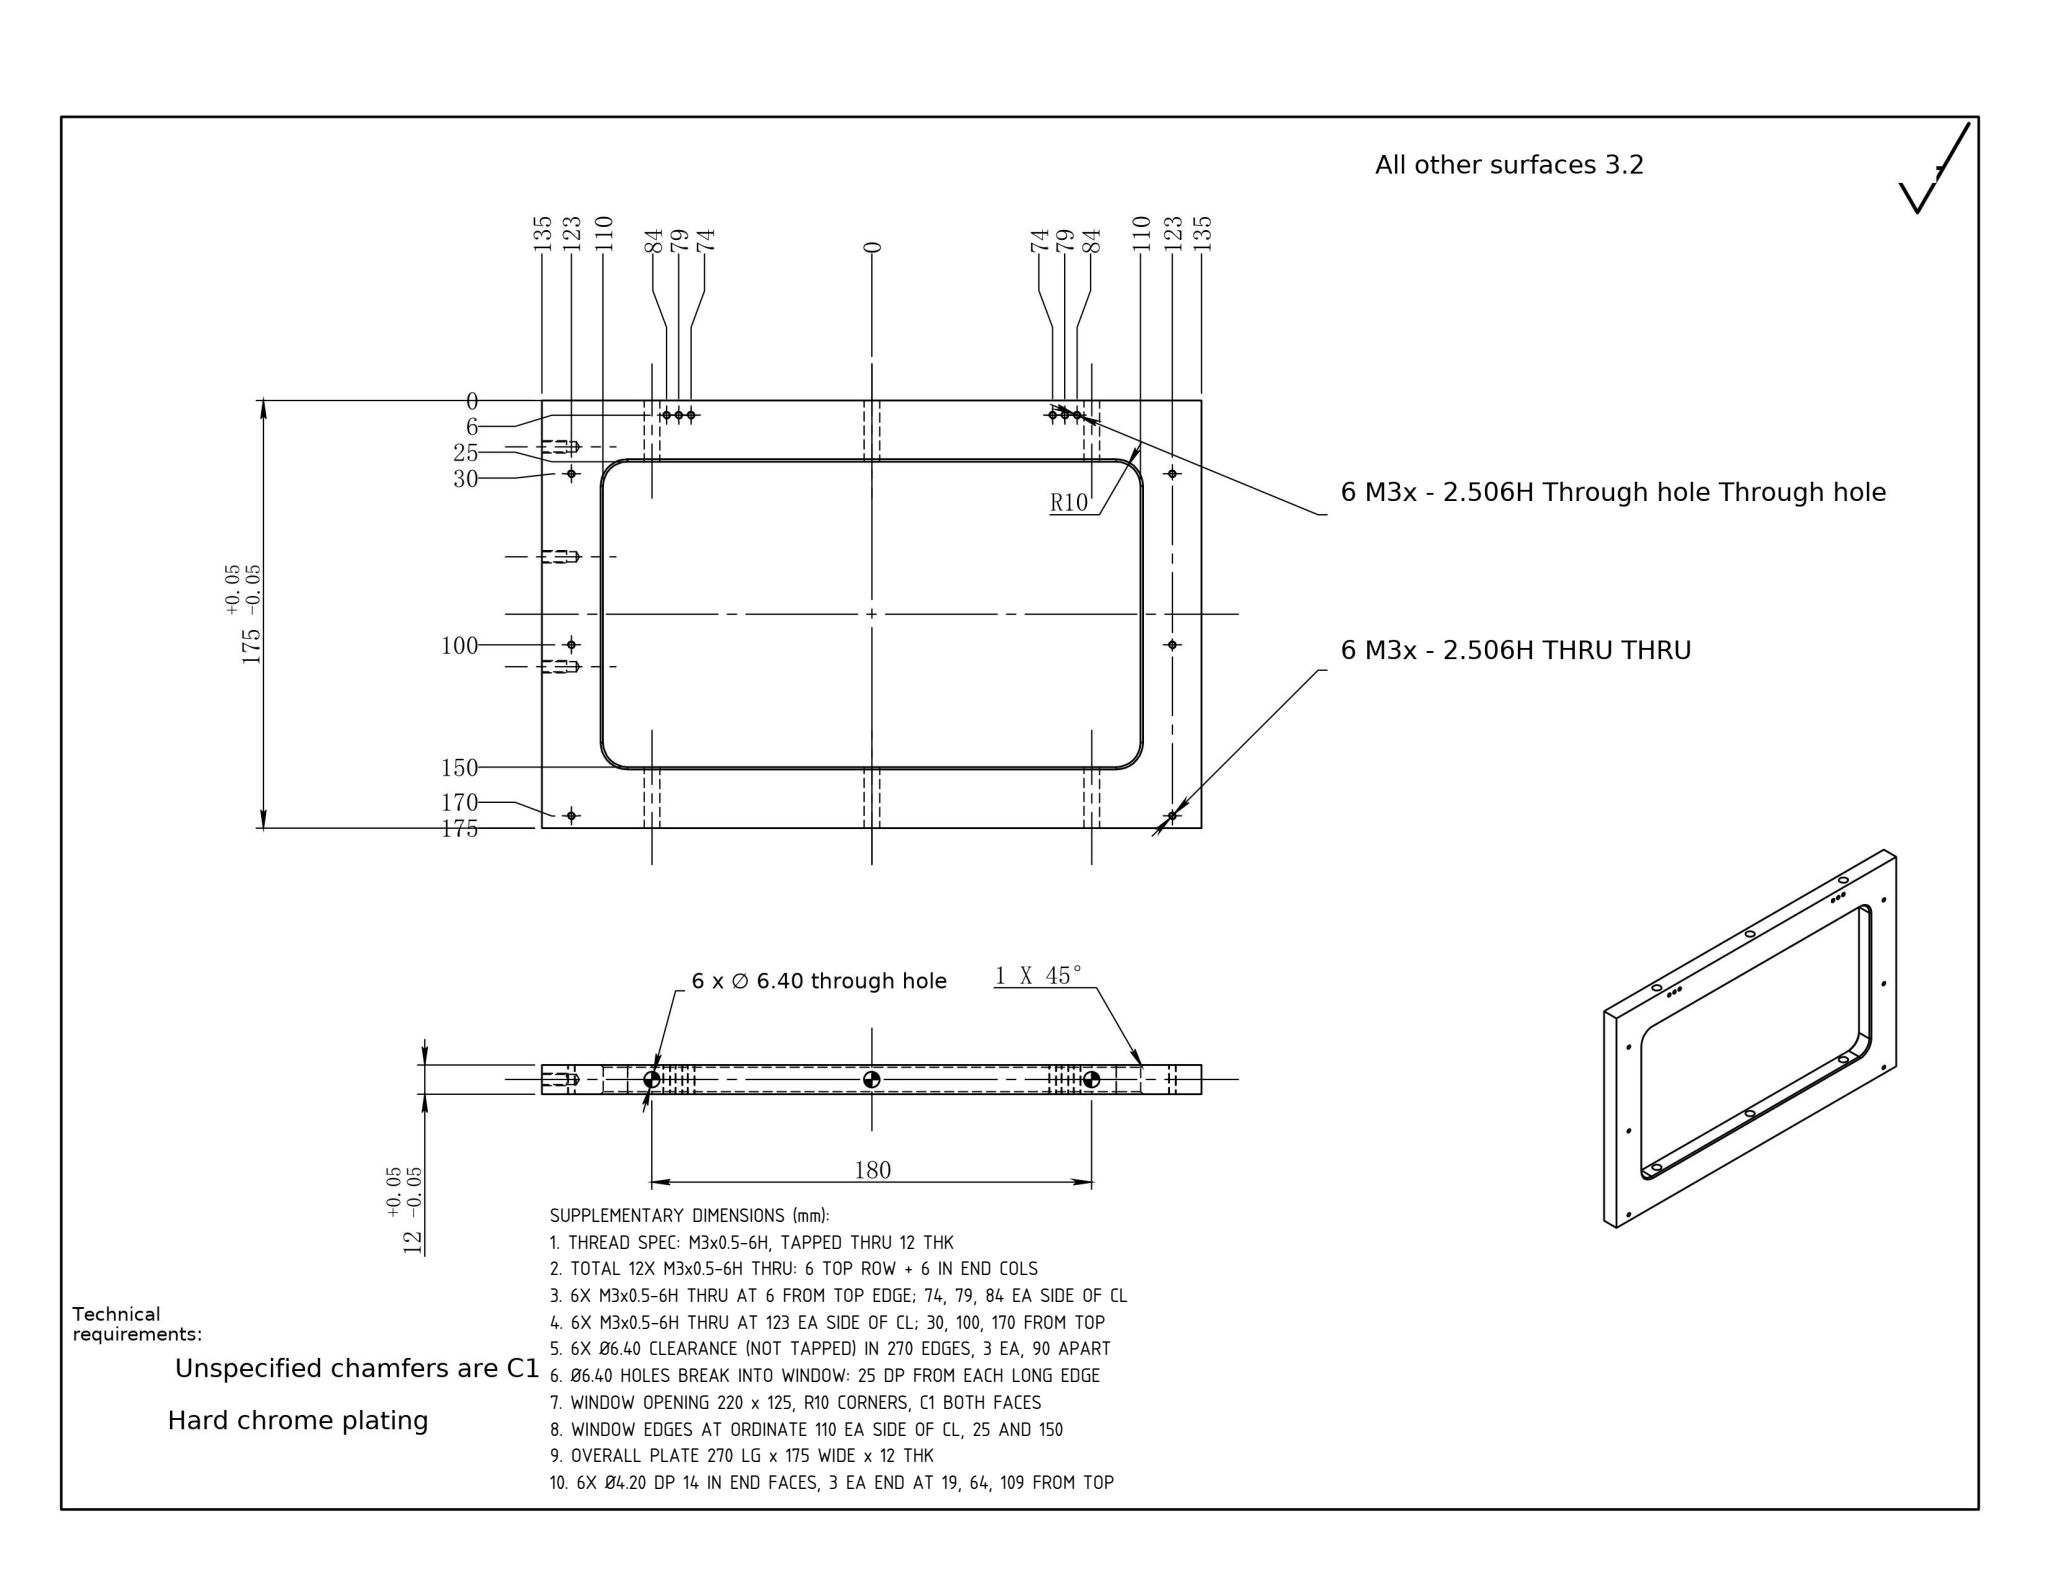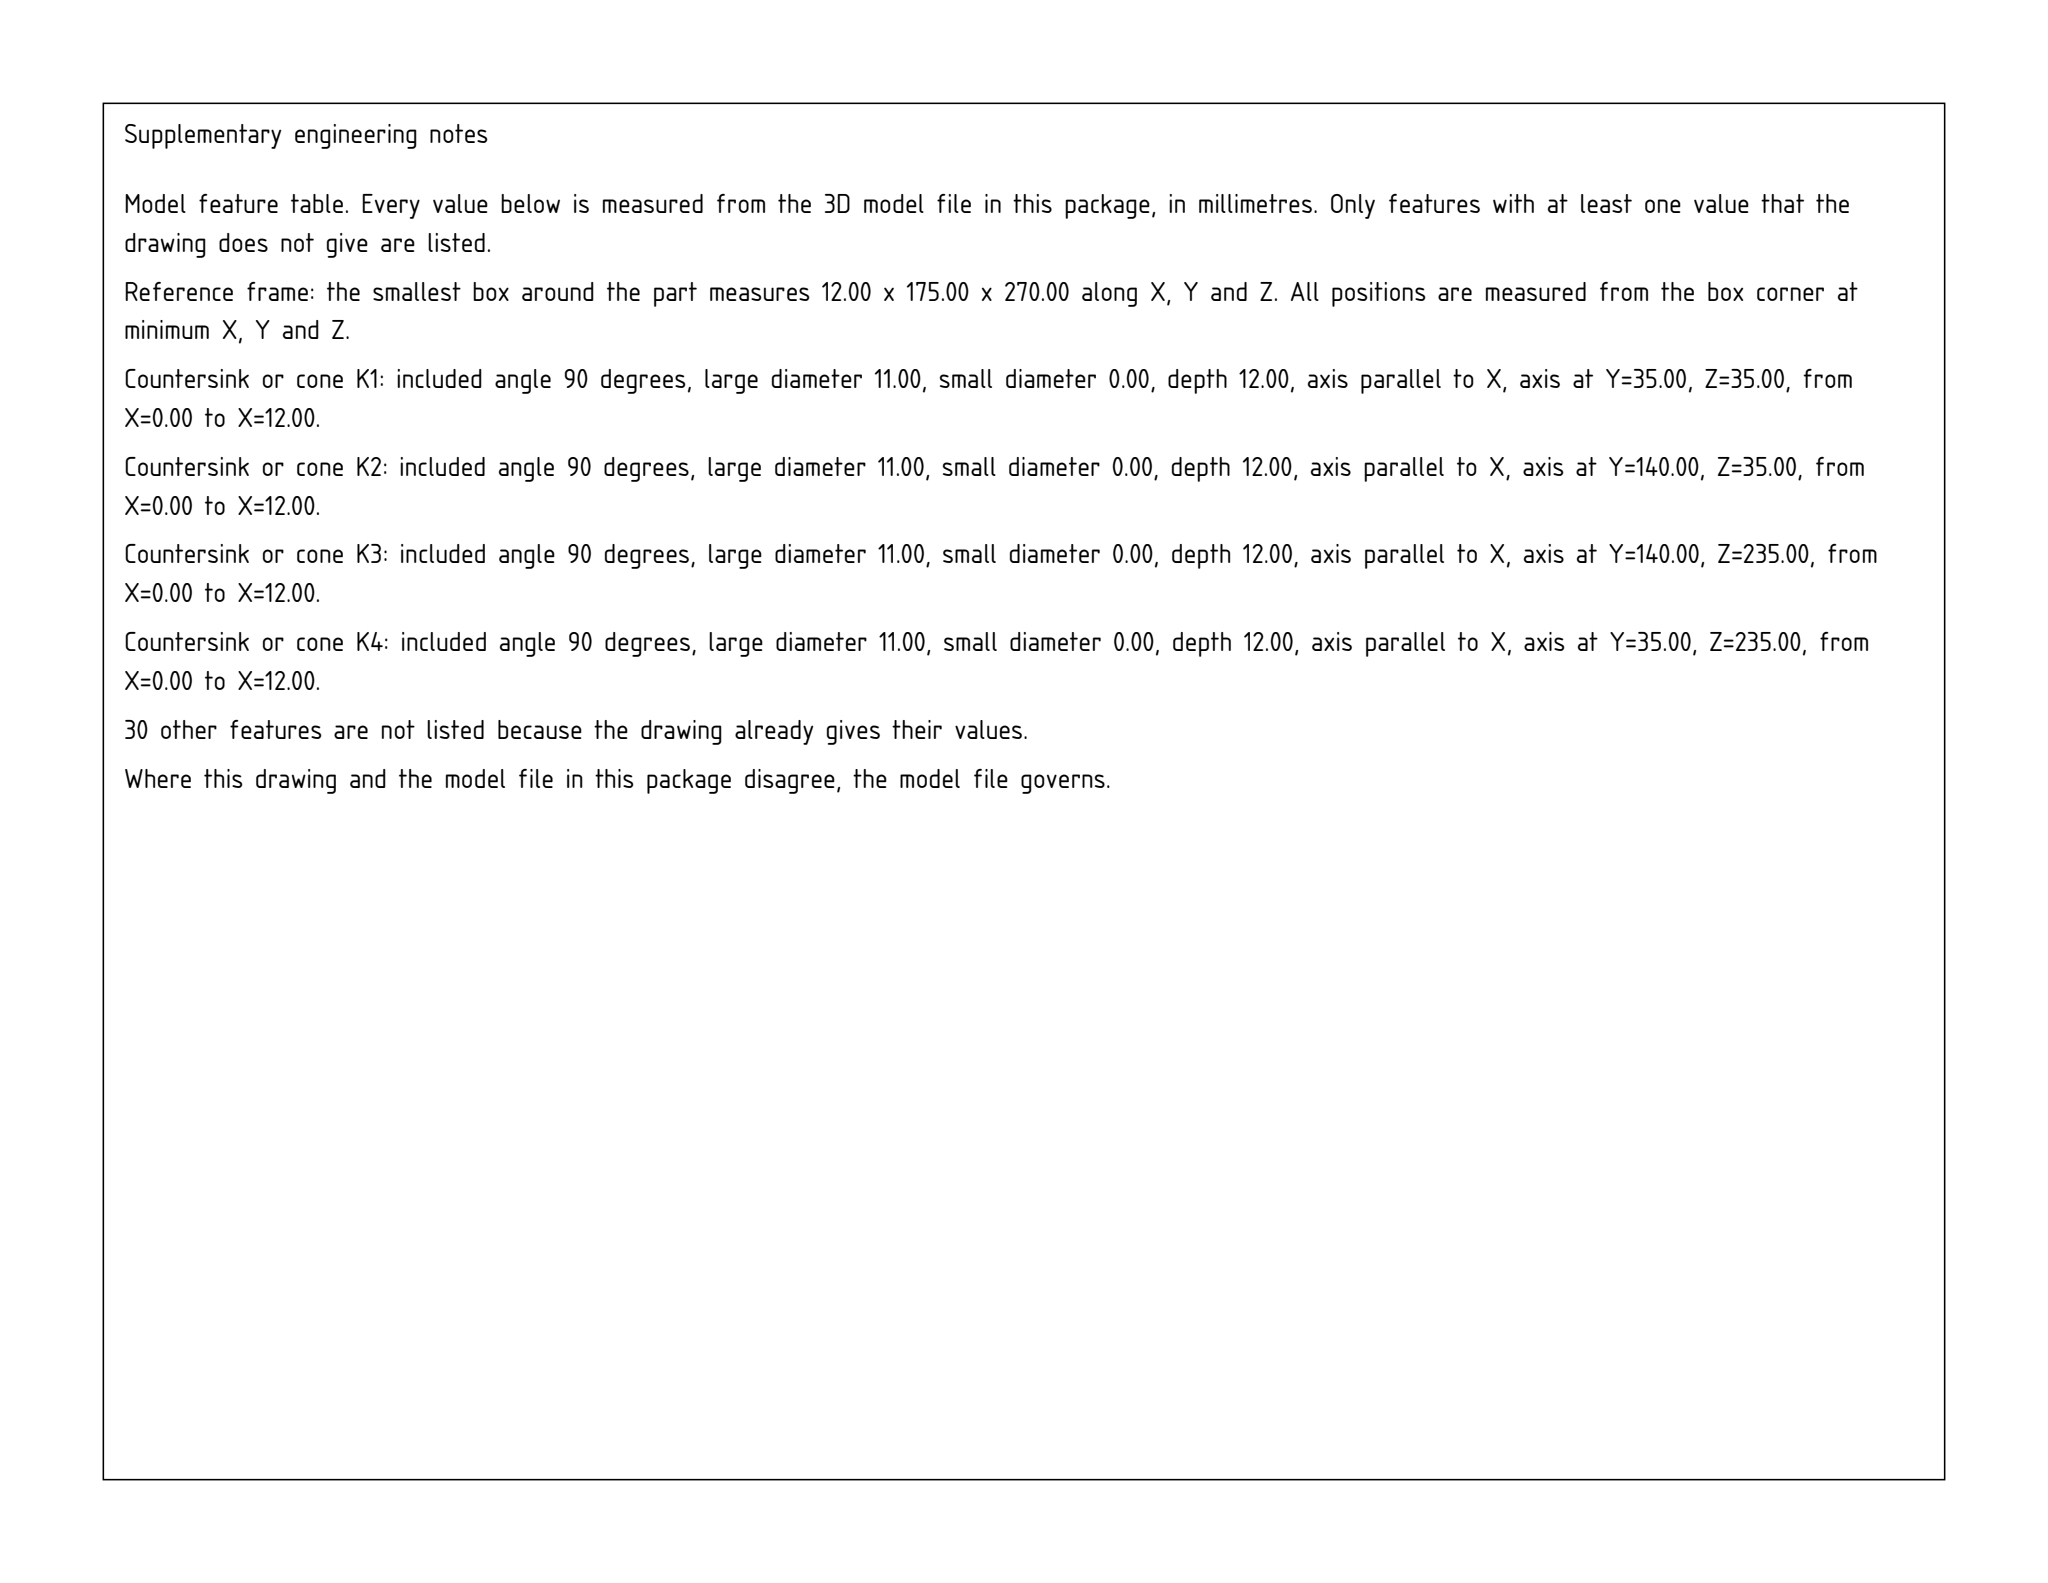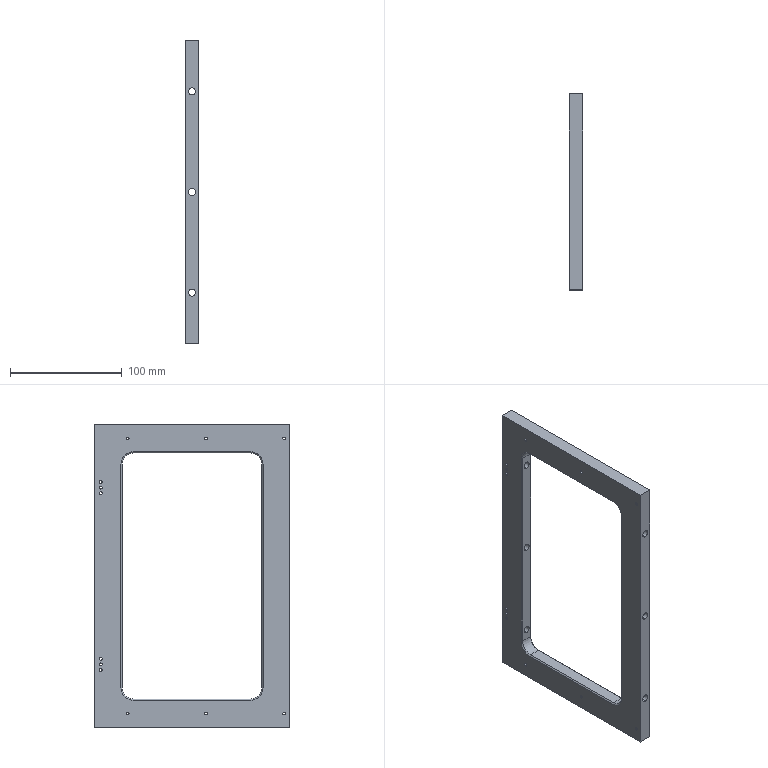Part | SolidWorks | mm | 1 solid | 78 faces | box 12 x 175 x 270 mm | volume 231223 mm3 | cylinder 46 | plane 18 | cone 14 | commonest cylinder face diameters 2.5 x24 6.4 x12 4.2 x6 20 x4
build123d program:
from build123d import *

# Parameters (mm, degrees)
SKETCH1_W                      = 12
SKETCH1_H                      = 270
BOSS_EXTRUDE1_DEPTH            = 87.5
SKETCH2_W                      = 220
SKETCH2_H                      = 125
CUT_EXTRUDE1_DEPTH             = 162.323
F_6_4_6_4_DIAMETER_HOLE1_D     = 6.4
F_6_4_6_4_DIAMETER_HOLE1_DEPTH = 25
FILLET1_R                      = 10
CHAMFER1_SIZE                  = 1
M5_TAPPED_HOLE1_D              = 4.2
M5_TAPPED_HOLE1_DEPTH          = 14
M5_TAPPED_HOLE1_TIP            = 1.262
M3_TAPPED_HOLE2_D              = 2.5
M3_TAPPED_HOLE1_D              = 2.5
LPATTERN1_COUNT                = 3
LPATTERN1_PITCH                = 70
MIRROR2_COPY_1_D               = 2.5
MIRROR2_COPY_2_D               = 2.5


with BuildPart() as part:
    # Sketch1 → Boss-Extrude1 (new, symmetric)
    with BuildSketch(Plane(origin=(0, 0, 0), x_dir=(1, 0, 0), z_dir=(0, 1, 0))):
        Rectangle(SKETCH1_W, SKETCH1_H)
    extrude(amount=BOSS_EXTRUDE1_DEPTH, both=True)

    # Sketch2 → Cut-Extrude1 (cut, through all)
    with BuildSketch(Plane(origin=(6, 0, 0), x_dir=(0, 0, -1), z_dir=(1, 0, 0))):
        Rectangle(SKETCH2_W, SKETCH2_H)
    extrude(amount=-CUT_EXTRUDE1_DEPTH, mode=Mode.SUBTRACT)

    # 6.4 _6.4_ Diameter Hole1
    with Locations(Plane(origin=(0, -62.5, 0), x_dir=(1, 0, 0), z_dir=(0, 1, 0))):
        with Locations((0, 0), (0, 90), (0, -90)):
            f_6_4_6_4_diameter_hole1 = Hole(F_6_4_6_4_DIAMETER_HOLE1_D / 2, depth=F_6_4_6_4_DIAMETER_HOLE1_DEPTH)

    # Fillet1
    fillet1_edges = [part.edges().sort_by_distance(p)[0] for p in [
        (0, 62.5, -110),
        (0, -62.5, -110),
        (0, -62.5, 110),
        (0, 62.5, 110),
    ]]
    fillet(fillet1_edges, radius=FILLET1_R)

    # Mirror1: 6.4 _6.4_ Diameter Hole1 across plane
    add(f_6_4_6_4_diameter_hole1.mirror(Plane.ZX), mode=Mode.SUBTRACT)

    # Chamfer1
    chamfer1_edges = [part.edges().sort_by_distance(p)[0] for p in [
        (6, 62.5, 0),
        (-6, 62.5, 0),
        (6, 0, -110),
        (-6, 0, -110),
        (6, 0, 110),
        (-6, 0, 110),
        (6, -62.5, 0),
        (-6, -62.5, 0),
        (6, 59.571, -107.071),
        (-6, 59.571, -107.071),
        (6, 59.571, 107.071),
        (-6, 59.571, 107.071),
        (6, -59.571, -107.071),
        (-6, -59.571, -107.071),
        (6, -59.571, 107.071),
        (-6, -59.571, 107.071),
    ]]
    chamfer(chamfer1_edges, length=CHAMFER1_SIZE)

    # M5 Tapped Hole1
    with Locations(Plane(origin=(0, 0, -135), x_dir=(-1, 0, 0), z_dir=(0, 0, -1))):
        with Locations((0, -21.5), (0, 23.5), (0, 68.5)):
            Hole(M5_TAPPED_HOLE1_D / 2, depth=M5_TAPPED_HOLE1_DEPTH)
            with Locations((0, 0, -(M5_TAPPED_HOLE1_DEPTH + M5_TAPPED_HOLE1_TIP / 2))):  # 118° drill point
                Cone(0, M5_TAPPED_HOLE1_D / 2, M5_TAPPED_HOLE1_TIP, mode=Mode.SUBTRACT)

    # M3 Tapped Hole2 (through all)
    with Locations(Plane(origin=(6, 0, 0), x_dir=(0, 0, -1), z_dir=(1, 0, 0))):
        with Locations((-84, 81.5), (-79, 81.5), (-74, 81.5)):
            m3_tapped_hole2 = Hole(M3_TAPPED_HOLE2_D / 2)

    # M3 Tapped Hole1 (through all)
    with Locations(Plane(origin=(6, 0, 0), x_dir=(0, 0, -1), z_dir=(1, 0, 0))):
        with Locations((-123, 57.5)):
            m3_tapped_hole1 = Hole(M3_TAPPED_HOLE1_D / 2)

    # LPattern1: M3 Tapped Hole1 ×3
    with Locations(*[(0, -i * LPATTERN1_PITCH, 0) for i in range(1, LPATTERN1_COUNT)]):
        add(m3_tapped_hole1, mode=Mode.SUBTRACT)

    # Mirror2: M3 Tapped Hole2, M3 Tapped Hole1 across plane
    add(m3_tapped_hole2.mirror(Plane.XY), mode=Mode.SUBTRACT)
    add(m3_tapped_hole1.mirror(Plane.XY), mode=Mode.SUBTRACT)

    # Mirror2 copy 1 (through all)
    with Locations(Plane(origin=(6, -70, 0), x_dir=(0, 0, 1), z_dir=(1, 0, 0))):
        with Locations((-123, -57.5)):
            Hole(MIRROR2_COPY_1_D / 2)

    # Mirror2 copy 2 (through all)
    with Locations(Plane(origin=(6, -140, 0), x_dir=(0, 0, 1), z_dir=(1, 0, 0))):
        with Locations((-123, -57.5)):
            Hole(MIRROR2_COPY_2_D / 2)


solid = part.part